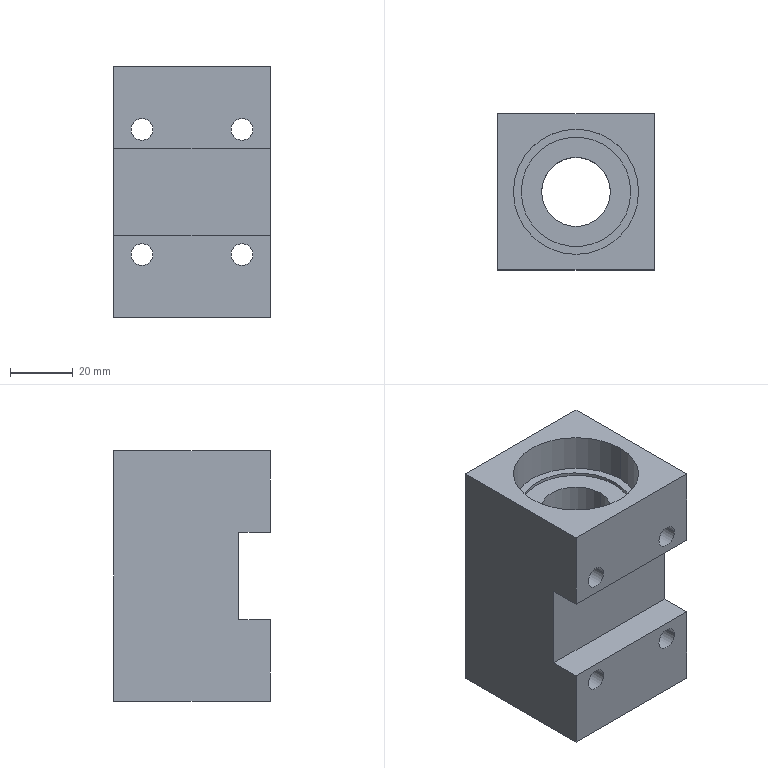Component | SolidWorks | PunchingAxisSeat-1 | 1 solid | 38 faces | box 50 x 50 x 80 mm | volume 125397 mm3 | cylinder 21 | plane 14 | cone 3 | commonest cylinder face diameters 7 x8 35 x5 40 x4 6.8 x2 22 x2
build123d program:
from build123d import *

# Parameters (mm, degrees)
SKETCH1_W             = 80
SKETCH1_H             = 50
EXTRUDE1_DEPTH        = 50
SKETCH2_R             = 11
EXTRUDE2_DEPTH        = 98.596
SKETCH3_R             = 20
EXTRUDE3_DEPTH        = 12
SKETCH4_R             = 17.5
EXTRUDE4_DEPTH        = 1
SKETCH5_W             = 28
SKETCH5_H             = 10
EXTRUDE5_DEPTH        = 69.739
SKETCH6_R             = 3.5
EXTRUDE6_DEPTH        = 82.24
M8_TAPPED_HOLE1_D     = 6.8
M8_TAPPED_HOLE1_DEPTH = 10
M8_TAPPED_HOLE1_TIP   = 2.043


with BuildPart() as part:
    # Sketch1 → Extrude1 (new body)
    with BuildSketch(Plane.XY):
        Rectangle(SKETCH1_W, SKETCH1_H)
    extrude(amount=EXTRUDE1_DEPTH)

    # Sketch2 → Extrude2 (cut, through all)
    with BuildSketch(Plane(origin=(40, 0, 0), x_dir=(0, 0, -1), z_dir=(1, 0, 0))):
        with Locations((-25, 0)):
            Circle(SKETCH2_R)
    extrude(amount=-EXTRUDE2_DEPTH, mode=Mode.SUBTRACT)

    # Sketch3 → Extrude3 (cut)
    with BuildSketch(Plane(origin=(40, 0, 0), x_dir=(0, 0, -1), z_dir=(1, 0, 0))):
        with Locations((-25, 0)):
            Circle(SKETCH3_R)
    extrude3 = extrude(amount=-EXTRUDE3_DEPTH, mode=Mode.SUBTRACT)

    # Sketch4 → Extrude4 (cut)
    with BuildSketch(Plane(origin=(28, 0, 0), x_dir=(0, 0, -1), z_dir=(1, 0, 0))):
        with Locations((-25, 0)):
            Circle(SKETCH4_R)
    extrude4 = extrude(amount=-EXTRUDE4_DEPTH, mode=Mode.SUBTRACT)

    # Mirror1: Extrude3, Extrude4 across plane
    add(extrude3.mirror(Plane(origin=(0, 0, 0), x_dir=(0, 0, 1), z_dir=(1, 0, 0))), mode=Mode.SUBTRACT)
    add(extrude4.mirror(Plane(origin=(0, 0, 0), x_dir=(0, 0, 1), z_dir=(1, 0, 0))), mode=Mode.SUBTRACT)

    # Sketch5 → Extrude5 (cut, through all)
    with BuildSketch(Plane.XY.offset(50)):
        with Locations((0, -20)):
            Rectangle(SKETCH5_W, SKETCH5_H)
    extrude(amount=-EXTRUDE5_DEPTH, mode=Mode.SUBTRACT)

    # Sketch6 → Extrude6 (cut, through all)
    with BuildSketch(Plane(origin=(0, 25, 0), x_dir=(1, 0, 0), z_dir=(0, 1, 0))):
        with Locations(Location((-20, -9, 0), (0, 0, 270))):
            Circle(SKETCH6_R)
        with Locations(Location((20, -9, 0), (0, 0, 270))):
            Circle(SKETCH6_R)
        with Locations(Location((-20, -41, 0), (0, 0, 270))):
            Circle(SKETCH6_R)
        with Locations(Location((20, -41, 0), (0, 0, 270))):
            Circle(SKETCH6_R)
    extrude(amount=-EXTRUDE6_DEPTH, mode=Mode.SUBTRACT)

    # M8 Tapped Hole1
    with Locations(Plane(origin=(0, 25, 0), x_dir=(-1, 0, 0), z_dir=(0, 1, 0))):
        with Locations((-30, 35)):
            Hole(M8_TAPPED_HOLE1_D / 2, depth=M8_TAPPED_HOLE1_DEPTH)
            with Locations((0, 0, -(M8_TAPPED_HOLE1_DEPTH + M8_TAPPED_HOLE1_TIP / 2))):  # 118° drill point
                Cone(0, M8_TAPPED_HOLE1_D / 2, M8_TAPPED_HOLE1_TIP, mode=Mode.SUBTRACT)


solid = part.part

# Placed as in the assembly
solid = solid.moved(Location((-235.944, 573.983, 197.789), (0, 90, 0)))